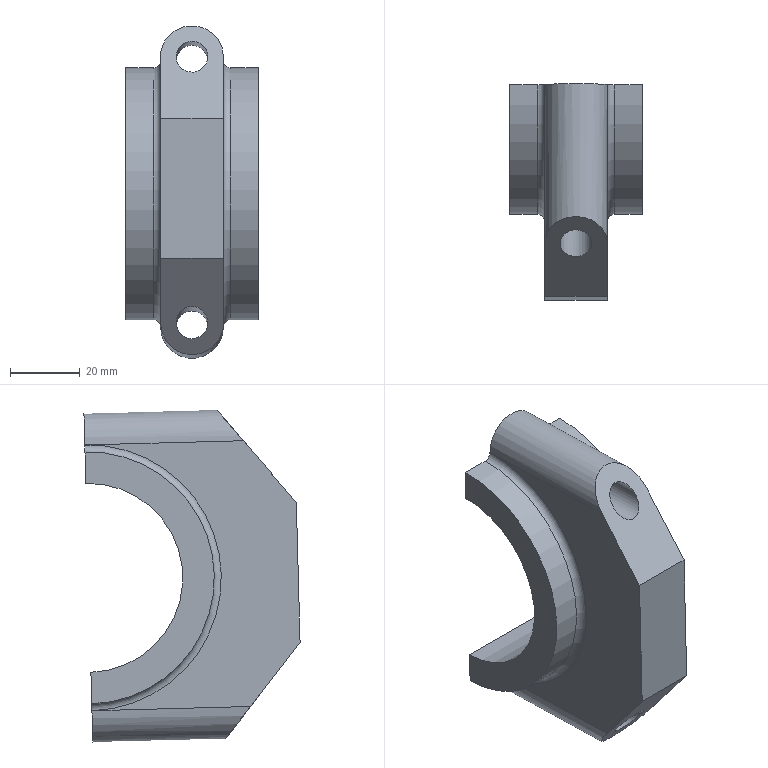Component | NX | 5_CONNECTING_ROD_CAP_2 | 1 solid | 18 faces | volume 79701 mm3 | plane 9 | cylinder 7 | torus 2 | commonest cylinder face diameters 72 x2 9 x2 18 x2 54 x1